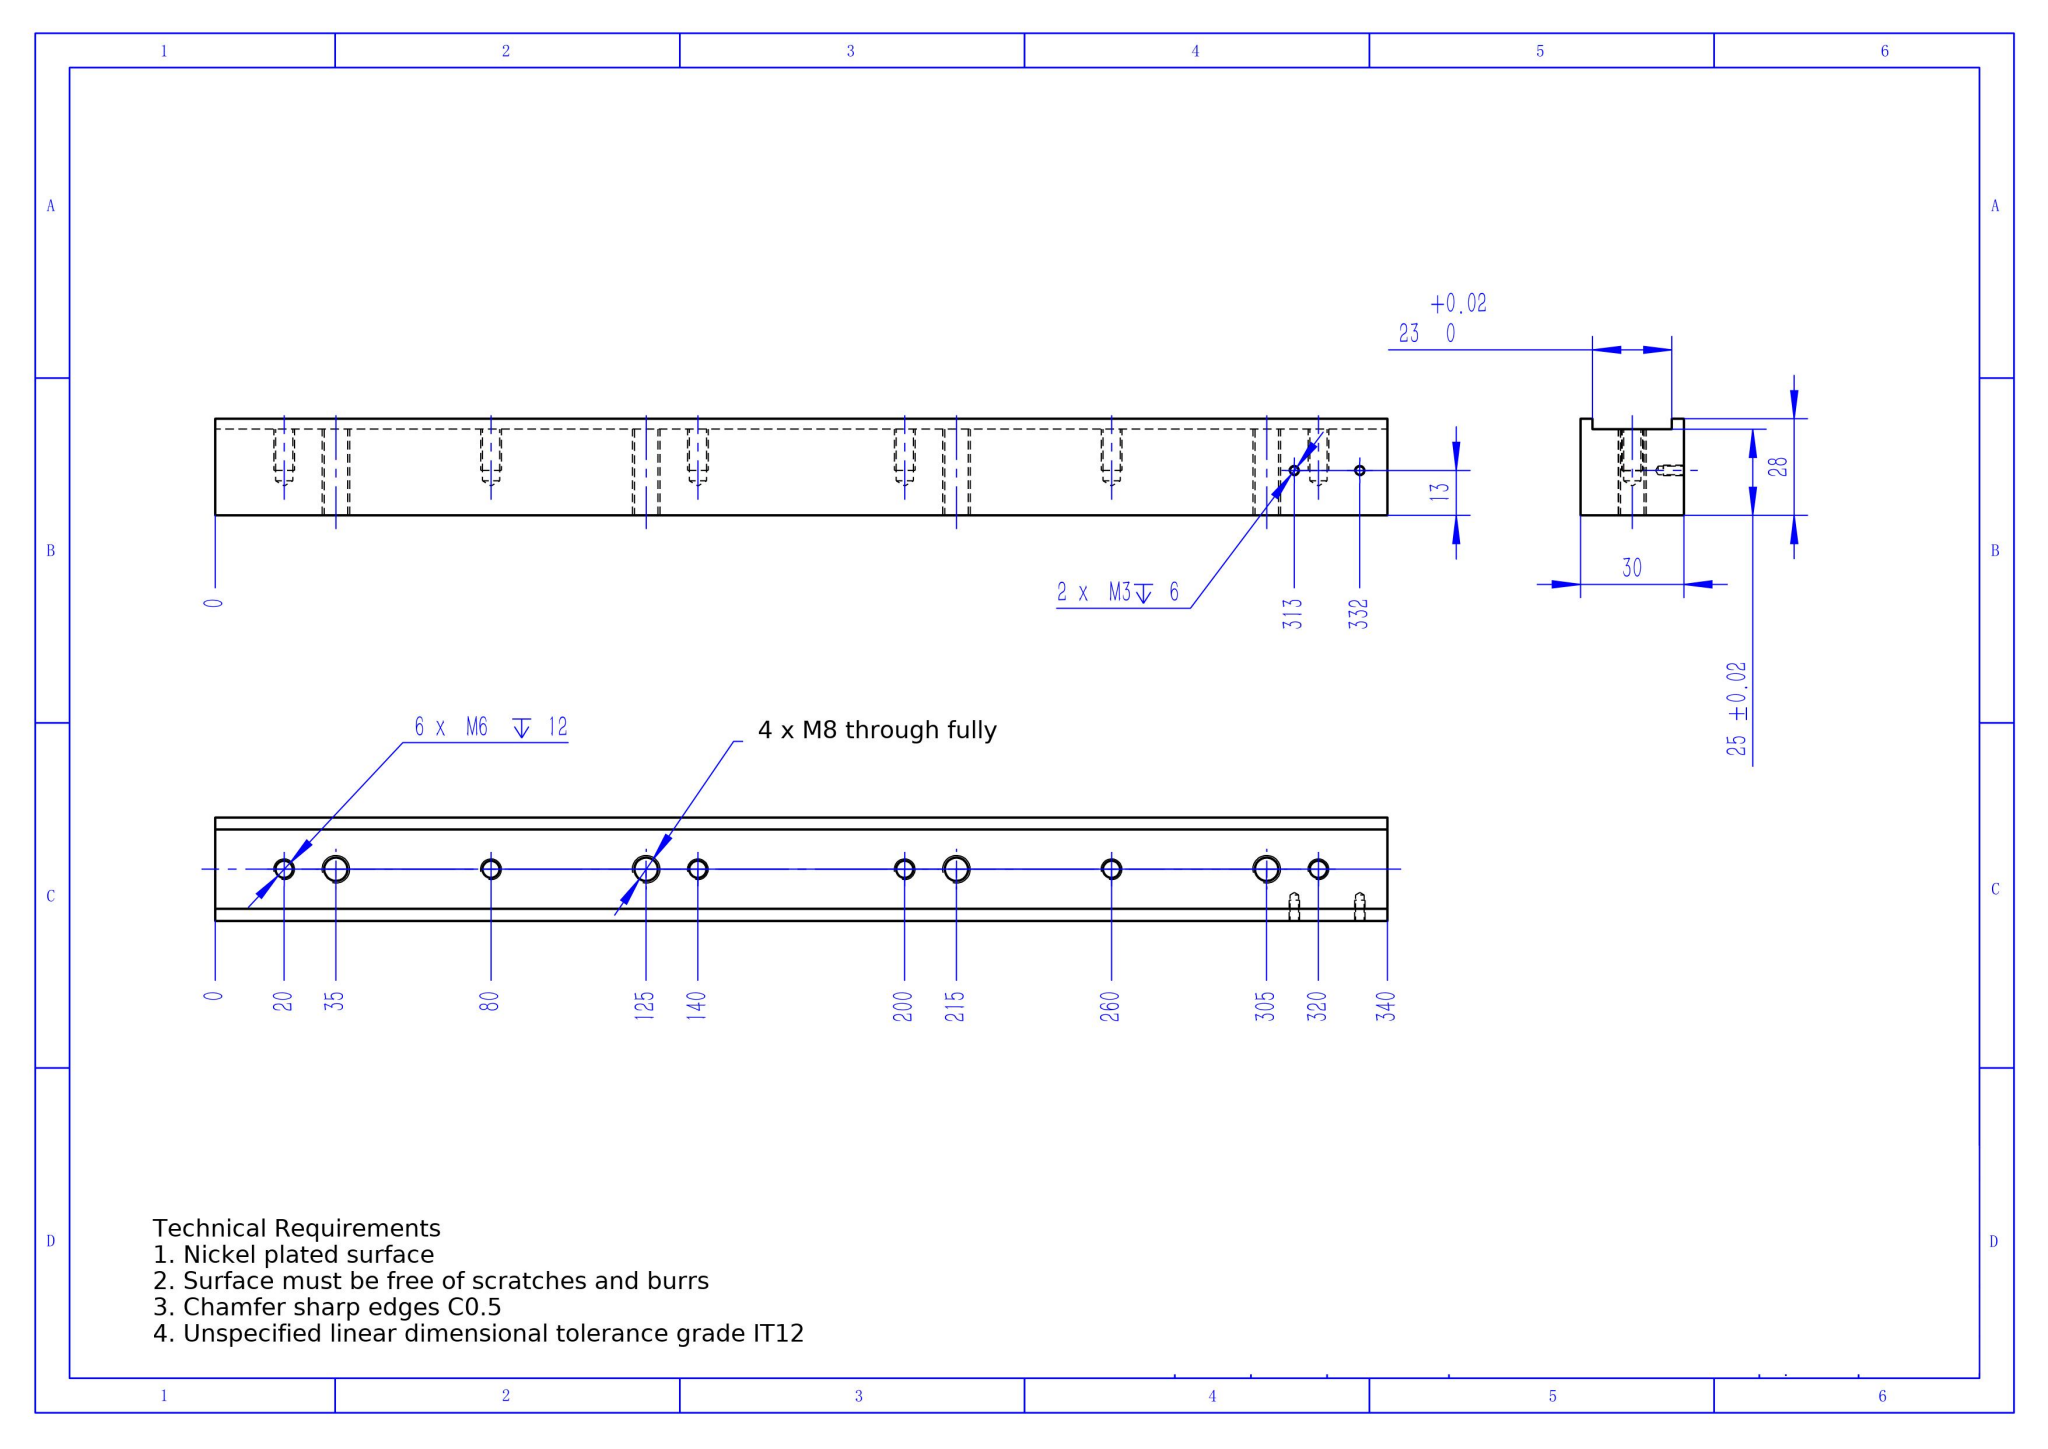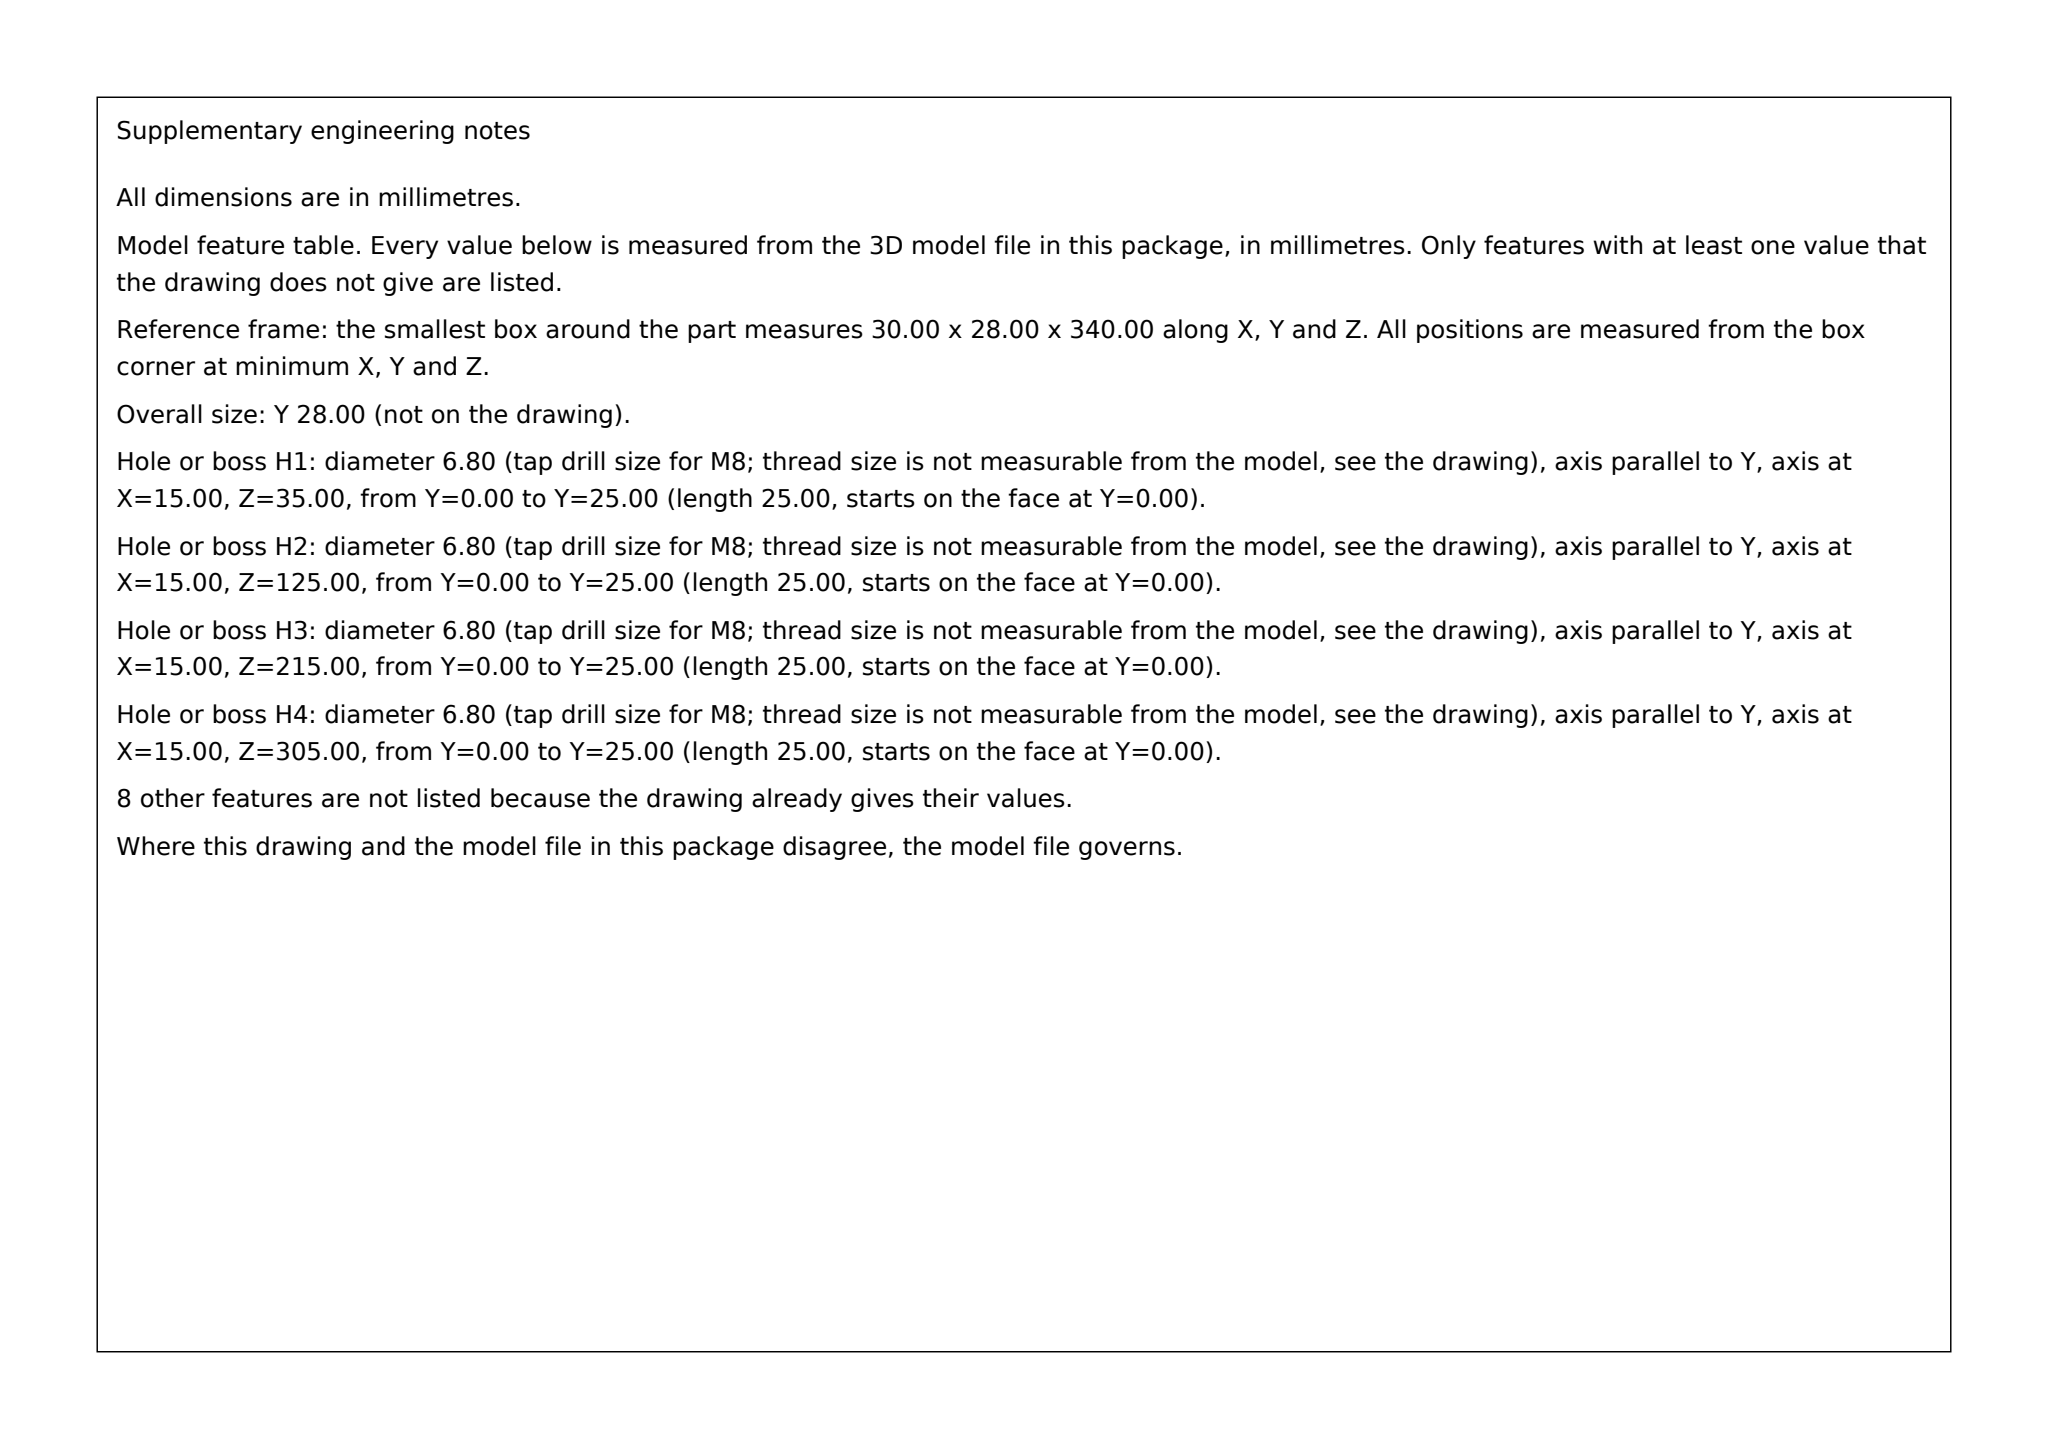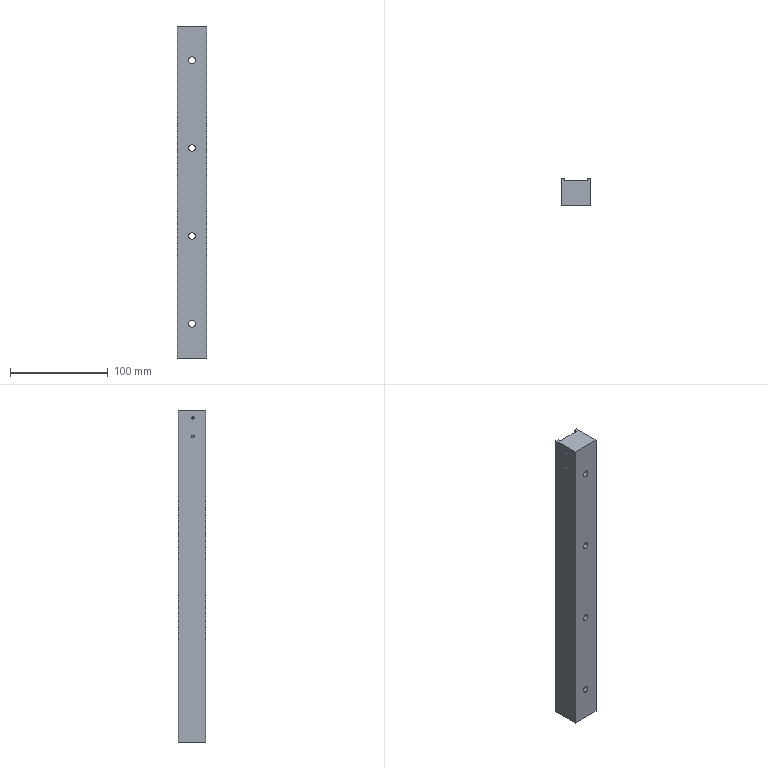Part | SolidWorks | mm | 1 solid | 50 faces | box 30 x 28 x 340 mm | volume 256606 mm3 | cylinder 24 | cone 16 | plane 10 | commonest cylinder face diameters 5 x12 6.8 x8 2.5 x4
build123d program:
from build123d import *

# Parameters (mm, degrees)
BOSS_EXTRUDE1_DEPTH   = 170
LPATTERN1_COUNT       = 6
LPATTERN1_PITCH       = 60
M8_TAPPED_HOLE1_D     = 6.8
LPATTERN2_COUNT       = 4
LPATTERN2_PITCH       = 90
M3_TAPPED_HOLE1_D     = 2.5
M3_TAPPED_HOLE1_DEPTH = 7.5
M3_TAPPED_HOLE1_TIP   = 0.7511


with BuildPart() as part:
    # Sketch1 → Boss-Extrude1 (new, symmetric)
    with BuildSketch(Plane.XY):
        Polygon((11.5, 28), (15, 28), (15, 0), (-15, 0), (-15, 28), (-11.5, 28), (-11.5, 25), (11.5, 25), align=None)
    extrude(amount=BOSS_EXTRUDE1_DEPTH, both=True)

    # Sketch3 → M6 Tapped Hole1 (revolve, cut)
    with BuildSketch(Plane(origin=(0, 25, 150), x_dir=(0, 0, 1), z_dir=(1, 0, 0))):
        Polygon((0, 0), (0, 16.502), (2.5, 15), (2.5, 0), align=None)
    m6_tapped_hole1 = revolve(axis=Axis((0, 31.35, 150), (0, -1, 0)), mode=Mode.SUBTRACT)

    # LPattern1: M6 Tapped Hole1 ×6
    with Locations(*[(0, 0, -i * LPATTERN1_PITCH) for i in range(1, LPATTERN1_COUNT)]):
        add(m6_tapped_hole1, mode=Mode.SUBTRACT)

    # M8 Tapped Hole1 (through all)
    with Locations(Plane(origin=(0, 0, 0), x_dir=(-1, 0, 0), z_dir=(0, -1, 0))):
        with Locations((0, 135)):
            m8_tapped_hole1 = Hole(M8_TAPPED_HOLE1_D / 2)

    # LPattern2: M8 Tapped Hole1 ×4
    with Locations(*[(0, 0, i * LPATTERN2_PITCH) for i in range(1, LPATTERN2_COUNT)]):
        add(m8_tapped_hole1, mode=Mode.SUBTRACT)

    # M3 Tapped Hole1
    with Locations(Plane.ZY.offset(15)):
        with Locations((162, 13), (143, 13)):
            Hole(M3_TAPPED_HOLE1_D / 2, depth=M3_TAPPED_HOLE1_DEPTH)
            with Locations((0, 0, -(M3_TAPPED_HOLE1_DEPTH + M3_TAPPED_HOLE1_TIP / 2))):  # 118° drill point
                Cone(0, M3_TAPPED_HOLE1_D / 2, M3_TAPPED_HOLE1_TIP, mode=Mode.SUBTRACT)


solid = part.part